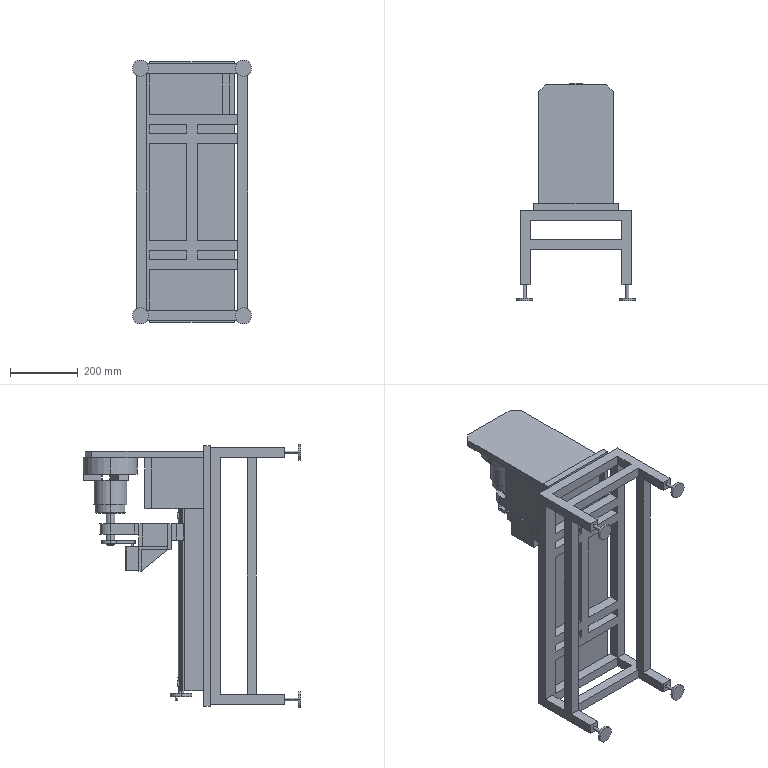Assembly | SolidWorks | mm | 18 component files | 43 solids | 658 faces | box 351.7 x 642.03 x 778.86 mm | volume 16917291 mm3 | plane 442 | cylinder 208 | cone 8 | commonest cylinder face diameters 5 x76 2 x40 10 x12 16 x10 48.35 x8 9.315 x8 25 x6 20 x6
Bill of materials:
BearingHousing | 1 |  | T-shaped flat bracket: a rectangular base bar with a perpendicular tab of the same thickness; the tab ends in a semicircle with one large through-hole, and the base bar has two smaller holes near its ends.
BearingHousingFloor | 1 |  | Open-top hollow rectangular box with thin walls. Two stacked flat tabs with round holes stick out from one side, the box has a stepped lower extension with an angled underside, and there is a small hole in one inner wall.
Belt | 1 |  | Thin-walled closed loop band with constant height and a teardrop or rounded-triangle outline: one large rounded end and one small rounded end joined by straight sides.
Chuck | 1 |  | Round disc with a small central through-hole. Underneath is a smaller stepped cylindrical boss carrying split prongs with chamfered, barbed tips around the central bore.
ChuckHolder | 1 |  | Thin, tall rectangular plate with a perpendicular thin flange at the top and a rectangular block under the flange. The front outline has chamfered top corners and a slightly wider lip at the bottom; small tabs project from the back face.
Frame | 1 |  | Rectangular open frame made of square-section bars, with intermediate horizontal cross members and a central vertical member. Four round foot pads on short cylindrical stems sit at the corners on one side.
GuideRail | 1 |  | Long straight extruded bar with a profiled cross-section: a rectangular body with rounded corners and symmetric V-shaped side notches, plus a row of small, evenly spaced holes along its length.
LeadScrew | 1 |  | Long slender round rod with a stepped profile: a longer main diameter section and a shorter reduced-diameter section at each end.
MirrorGuideRail | 1 |  | Long straight extruded bar with a profiled cross-section: a rectangular body with rounded corners and symmetric V-shaped side notches, plus a row of small, evenly spaced holes along its length.
MirrorSlider | 1 |  | Rectangular prismatic block with a channel through its length. The channel is open on one face and has a profiled cross-section with rounded corners and inclined undercut flanks.
Motor | 1 |  | Square-section prismatic body with slightly rounded vertical edges. One end face has a shallow raised circular boss, and a smaller cylindrical shaft sticks out from the centre of the boss.
PolishingAxis | 1 |  | Short stepped cylindrical pin: a main body with a slightly larger-diameter collar band near one end and chamfered ends.
PolishingHead | 1 |  | Flat cylindrical disc with a small central through-hole and a chamfer around one outer edge (washer- or spacer-like shape).
Pulley | 1 |  | Flat ring/washer-like annulus with a large central through-hole and plain square edges.
RockerArm | 1 |  | Flat disc with a central through-hole and one small tapered (conical) peg sticking out of one face, offset from the central axis.
Slider | 1 |  | Rectangular prismatic block with a stepped channel of constant cross-section running its full length. The channel is open on one long face and has symmetric stepped, angled side walls with rounded corners.
SmallWheel | 1 |  | Thick-walled cylindrical sleeve/spacer with a concentric central through-bore and flat end faces.
Workpiece | 1 |  | Thin-walled, open-ended cylindrical tube or ring with flat ends.
Mates:
1. coincident | Pulley-1 face at (0, 0, -195) dir (0, 0, 1) | SmallWheel-1 face at (48.507, -64.609, -195) dir (0, 0, 1)
2. coincident | BearingHousingFloor-1 face at (0, -84.609, -146) dir (0, 1, 0) | Motor-1 face at (-11.374, -84.609, -171.311) dir (0, -1, 0)
3. coincident | BearingHousingFloor-1 face at (68.507, -84.609, -223.341) dir (1, 0, 0) | Motor-1 face at (68.507, -84.609, -215) dir (1, 0, 0)